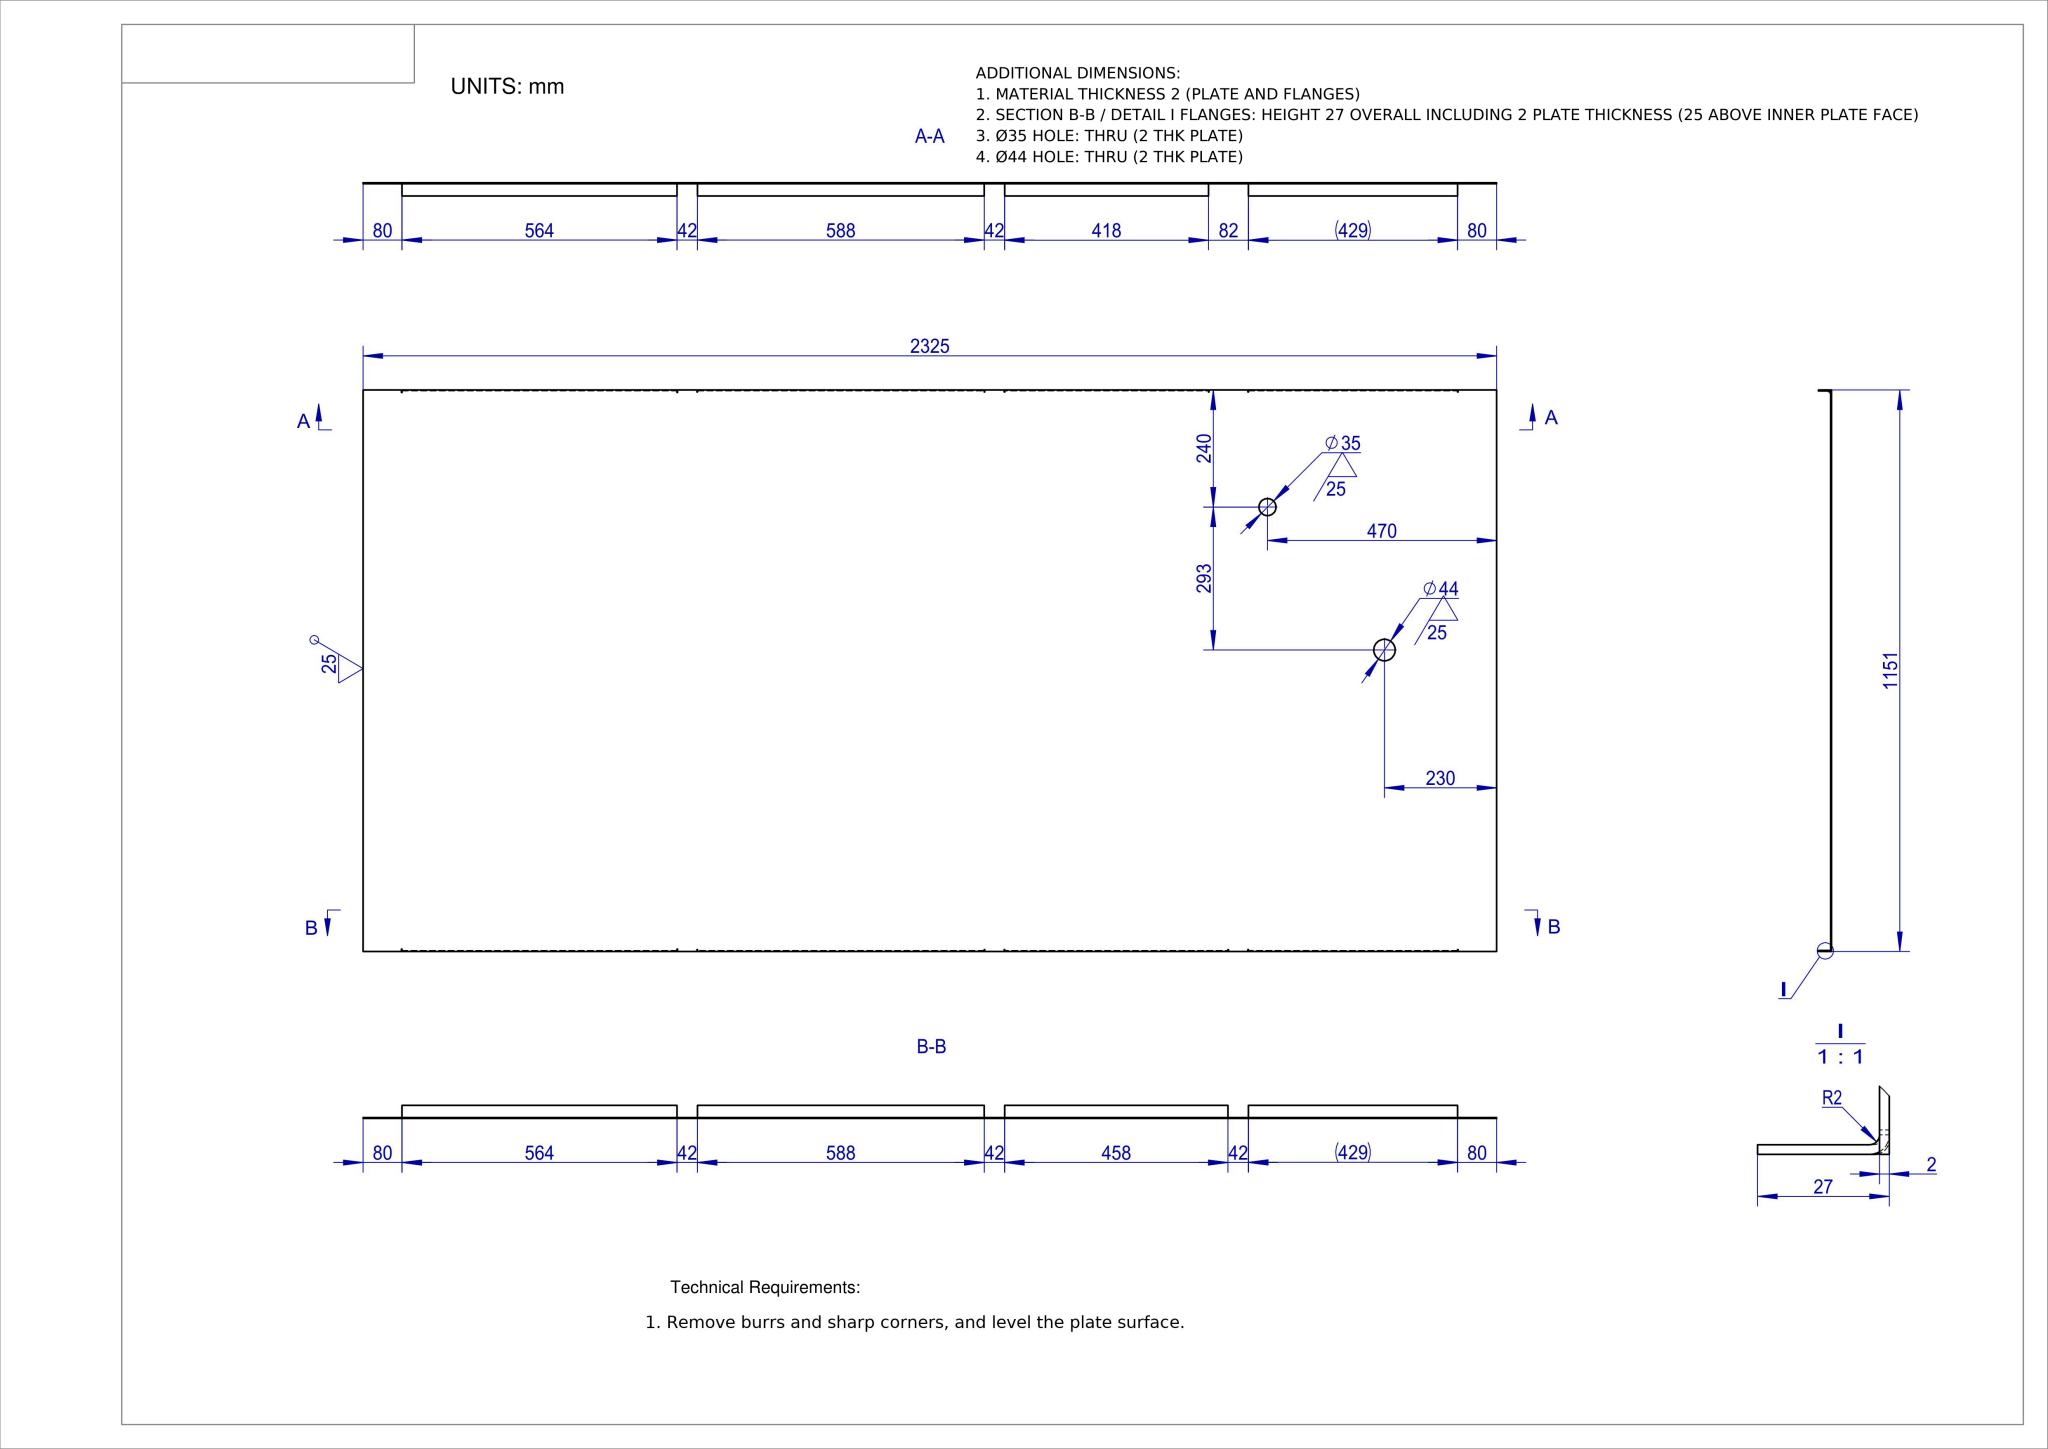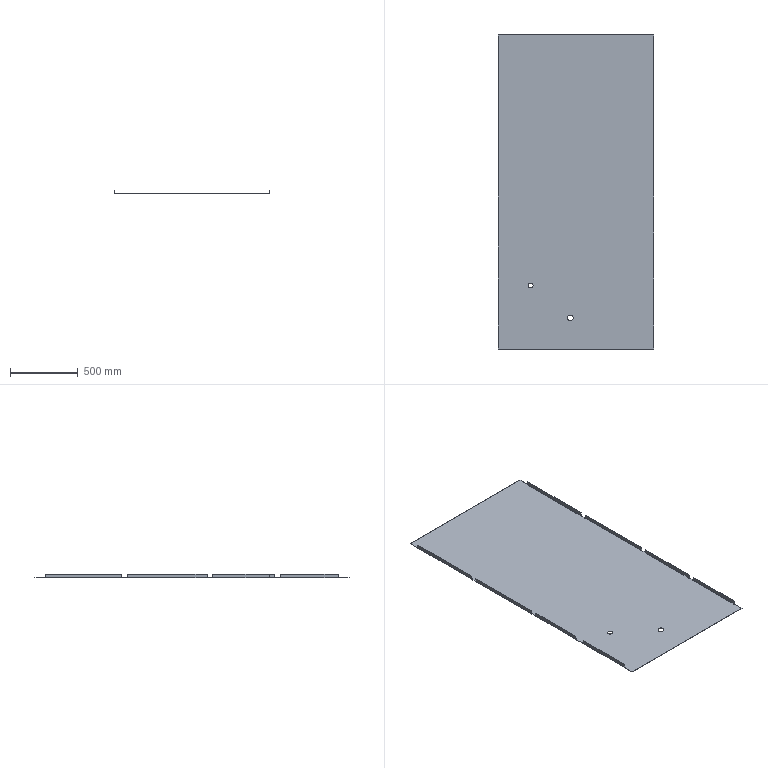Part | NX | mm | 1 solid | 138 faces | box 1151 x 2325 x 27 mm | volume 5541048 mm3 | plane 118 | cylinder 20 | commonest cylinder face diameters 6 x6 2 x6 35 x2 44 x2 8 x2 4 x2